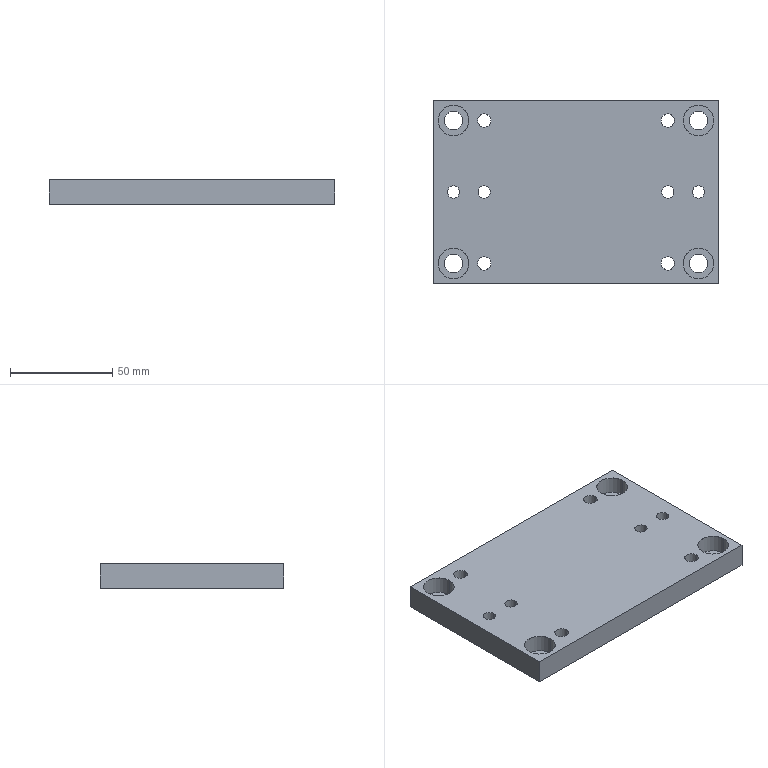Component | SolidWorks | Y-AxisSliderShimPlate-1 | 1 solid | 102 faces | box 140 x 90 x 12 mm | volume 139699 mm3 | cone 48 | cylinder 40 | plane 14 | commonest cylinder face diameters 15 x8 9 x8 6 x8 11 x8 6.6 x8
build123d program:
from build123d import *

# Parameters (mm, degrees)
SKETCH1_W                                      = 140
SKETCH1_H                                      = 90
BOSS_EXTRUDE1_DEPTH                            = 12
SKETCH2_R                                      = 3
CUT_EXTRUDE1_DEPTH                             = 85.077
M6_HEX_SOCKET_HEAD_CAP_SCREW_CBORE1_AT_2_COUNT = 2
M6_HEX_SOCKET_HEAD_CAP_SCREW_CBORE1_AT_2_PITCH = 70
M6_HEX_SOCKET_HEAD_CAP_SCREW_CBORE1_AT_3_COUNT = 2
M6_HEX_SOCKET_HEAD_CAP_SCREW_CBORE1_AT_3_PITCH = 114.018
M6_HEX_SOCKET_HEAD_CAP_SCREW_CBORE1_AT_4_COUNT = 2
M6_HEX_SOCKET_HEAD_CAP_SCREW_CBORE1_AT_4_PITCH = 90
SKETCH5_R                                      = 3
CUT_EXTRUDE2_DEPTH                             = 85.077
M8_HEX_SOCKET_HEAD_CAP_SCREW_CBORE1_AT_2_COUNT = 2
M8_HEX_SOCKET_HEAD_CAP_SCREW_CBORE1_AT_2_PITCH = 120
M8_HEX_SOCKET_HEAD_CAP_SCREW_CBORE1_AT_3_COUNT = 2
M8_HEX_SOCKET_HEAD_CAP_SCREW_CBORE1_AT_3_PITCH = 138.924
M8_HEX_SOCKET_HEAD_CAP_SCREW_CBORE1_AT_4_COUNT = 2
M8_HEX_SOCKET_HEAD_CAP_SCREW_CBORE1_AT_4_PITCH = 70


with BuildPart() as part:
    # Sketch1 → Boss-Extrude1 (new body)
    with BuildSketch(Plane.XY):
        Rectangle(SKETCH1_W, SKETCH1_H)
    extrude(amount=BOSS_EXTRUDE1_DEPTH)

    # Sketch2 → Cut-Extrude1 (cut, through all)
    with BuildSketch(Plane.XY.offset(12)):
        with Locations((-45, 0)):
            Circle(SKETCH2_R)
        with Locations((45, 0)):
            Circle(SKETCH2_R)
    extrude(amount=-CUT_EXTRUDE1_DEPTH, mode=Mode.SUBTRACT)

    # Sketch3 → M6 Hex Socket Head Cap Screw CBORE1 (revolve, cut)
    with BuildSketch(Plane(origin=(-45, 35, 12), x_dir=(0, -1, 0), z_dir=(1, 0, 0))):
        Polygon((0, 0), (0, 12), (3.325, 12), (3.3, 11.975), (3.3, 6.425), (3.325, 6.4), (5.5, 6.4), (5.5, 0.025), (5.525, 0), align=None)
    m6_hex_socket_head_cap_screw_cbore1 = revolve(axis=Axis((-45, 35, 18.35), (0, 0, -1)), mode=Mode.SUBTRACT)

    # M6 Hex Socket Head Cap Screw CBORE1 at 2: M6 Hex Socket Head Cap Screw CBORE1 ×2
    with Locations(*[(0, -i * M6_HEX_SOCKET_HEAD_CAP_SCREW_CBORE1_AT_2_PITCH, 0) for i in range(1, M6_HEX_SOCKET_HEAD_CAP_SCREW_CBORE1_AT_2_COUNT)]):
        add(m6_hex_socket_head_cap_screw_cbore1, mode=Mode.SUBTRACT)

    # M6 Hex Socket Head Cap Screw CBORE1 at 3: M6 Hex Socket Head Cap Screw CBORE1 ×2
    with Locations(*[Vector(0.7894, -0.6139, 0) * (i * M6_HEX_SOCKET_HEAD_CAP_SCREW_CBORE1_AT_3_PITCH) for i in range(1, M6_HEX_SOCKET_HEAD_CAP_SCREW_CBORE1_AT_3_COUNT)]):
        add(m6_hex_socket_head_cap_screw_cbore1, mode=Mode.SUBTRACT)

    # M6 Hex Socket Head Cap Screw CBORE1 at 4: M6 Hex Socket Head Cap Screw CBORE1 ×2
    with Locations(*[(i * M6_HEX_SOCKET_HEAD_CAP_SCREW_CBORE1_AT_4_PITCH, 0, 0) for i in range(1, M6_HEX_SOCKET_HEAD_CAP_SCREW_CBORE1_AT_4_COUNT)]):
        add(m6_hex_socket_head_cap_screw_cbore1, mode=Mode.SUBTRACT)

    # Sketch5 → Cut-Extrude2 (cut, through all)
    with BuildSketch(Plane(origin=(0, 0, 0), x_dir=(-1, 0, 0), z_dir=(0, 0, -1))):
        with Locations((-60, 0)):
            Circle(SKETCH5_R)
        with Locations((60, 0)):
            Circle(SKETCH5_R)
    extrude(amount=-CUT_EXTRUDE2_DEPTH, mode=Mode.SUBTRACT)

    # Sketch6 → M8 Hex Socket Head Cap Screw CBORE1 (revolve, cut)
    with BuildSketch(Plane(origin=(60, 35, 0), x_dir=(0, 1, 0), z_dir=(1, 0, 0))):
        Polygon((0, 0), (0, 12), (4.525, 12), (4.5, 11.975), (4.5, 8.625), (4.525, 8.6), (7.5, 8.6), (7.5, 0.025), (7.525, 0), align=None)
    m8_hex_socket_head_cap_screw_cbore1 = revolve(axis=Axis((60, 35, -6.35), (0, 0, 1)), mode=Mode.SUBTRACT)

    # M8 Hex Socket Head Cap Screw CBORE1 at 2: M8 Hex Socket Head Cap Screw CBORE1 ×2
    with Locations(*[(-i * M8_HEX_SOCKET_HEAD_CAP_SCREW_CBORE1_AT_2_PITCH, 0, 0) for i in range(1, M8_HEX_SOCKET_HEAD_CAP_SCREW_CBORE1_AT_2_COUNT)]):
        add(m8_hex_socket_head_cap_screw_cbore1, mode=Mode.SUBTRACT)

    # M8 Hex Socket Head Cap Screw CBORE1 at 3: M8 Hex Socket Head Cap Screw CBORE1 ×2
    with Locations(*[Vector(-0.8638, -0.5039, 0) * (i * M8_HEX_SOCKET_HEAD_CAP_SCREW_CBORE1_AT_3_PITCH) for i in range(1, M8_HEX_SOCKET_HEAD_CAP_SCREW_CBORE1_AT_3_COUNT)]):
        add(m8_hex_socket_head_cap_screw_cbore1, mode=Mode.SUBTRACT)

    # M8 Hex Socket Head Cap Screw CBORE1 at 4: M8 Hex Socket Head Cap Screw CBORE1 ×2
    with Locations(*[(0, -i * M8_HEX_SOCKET_HEAD_CAP_SCREW_CBORE1_AT_4_PITCH, 0) for i in range(1, M8_HEX_SOCKET_HEAD_CAP_SCREW_CBORE1_AT_4_COUNT)]):
        add(m8_hex_socket_head_cap_screw_cbore1, mode=Mode.SUBTRACT)


solid = part.part

# Placed as in the assembly
solid = solid.moved(Location((-28.271, -71.882, -86.5), (180, 0, 0)))